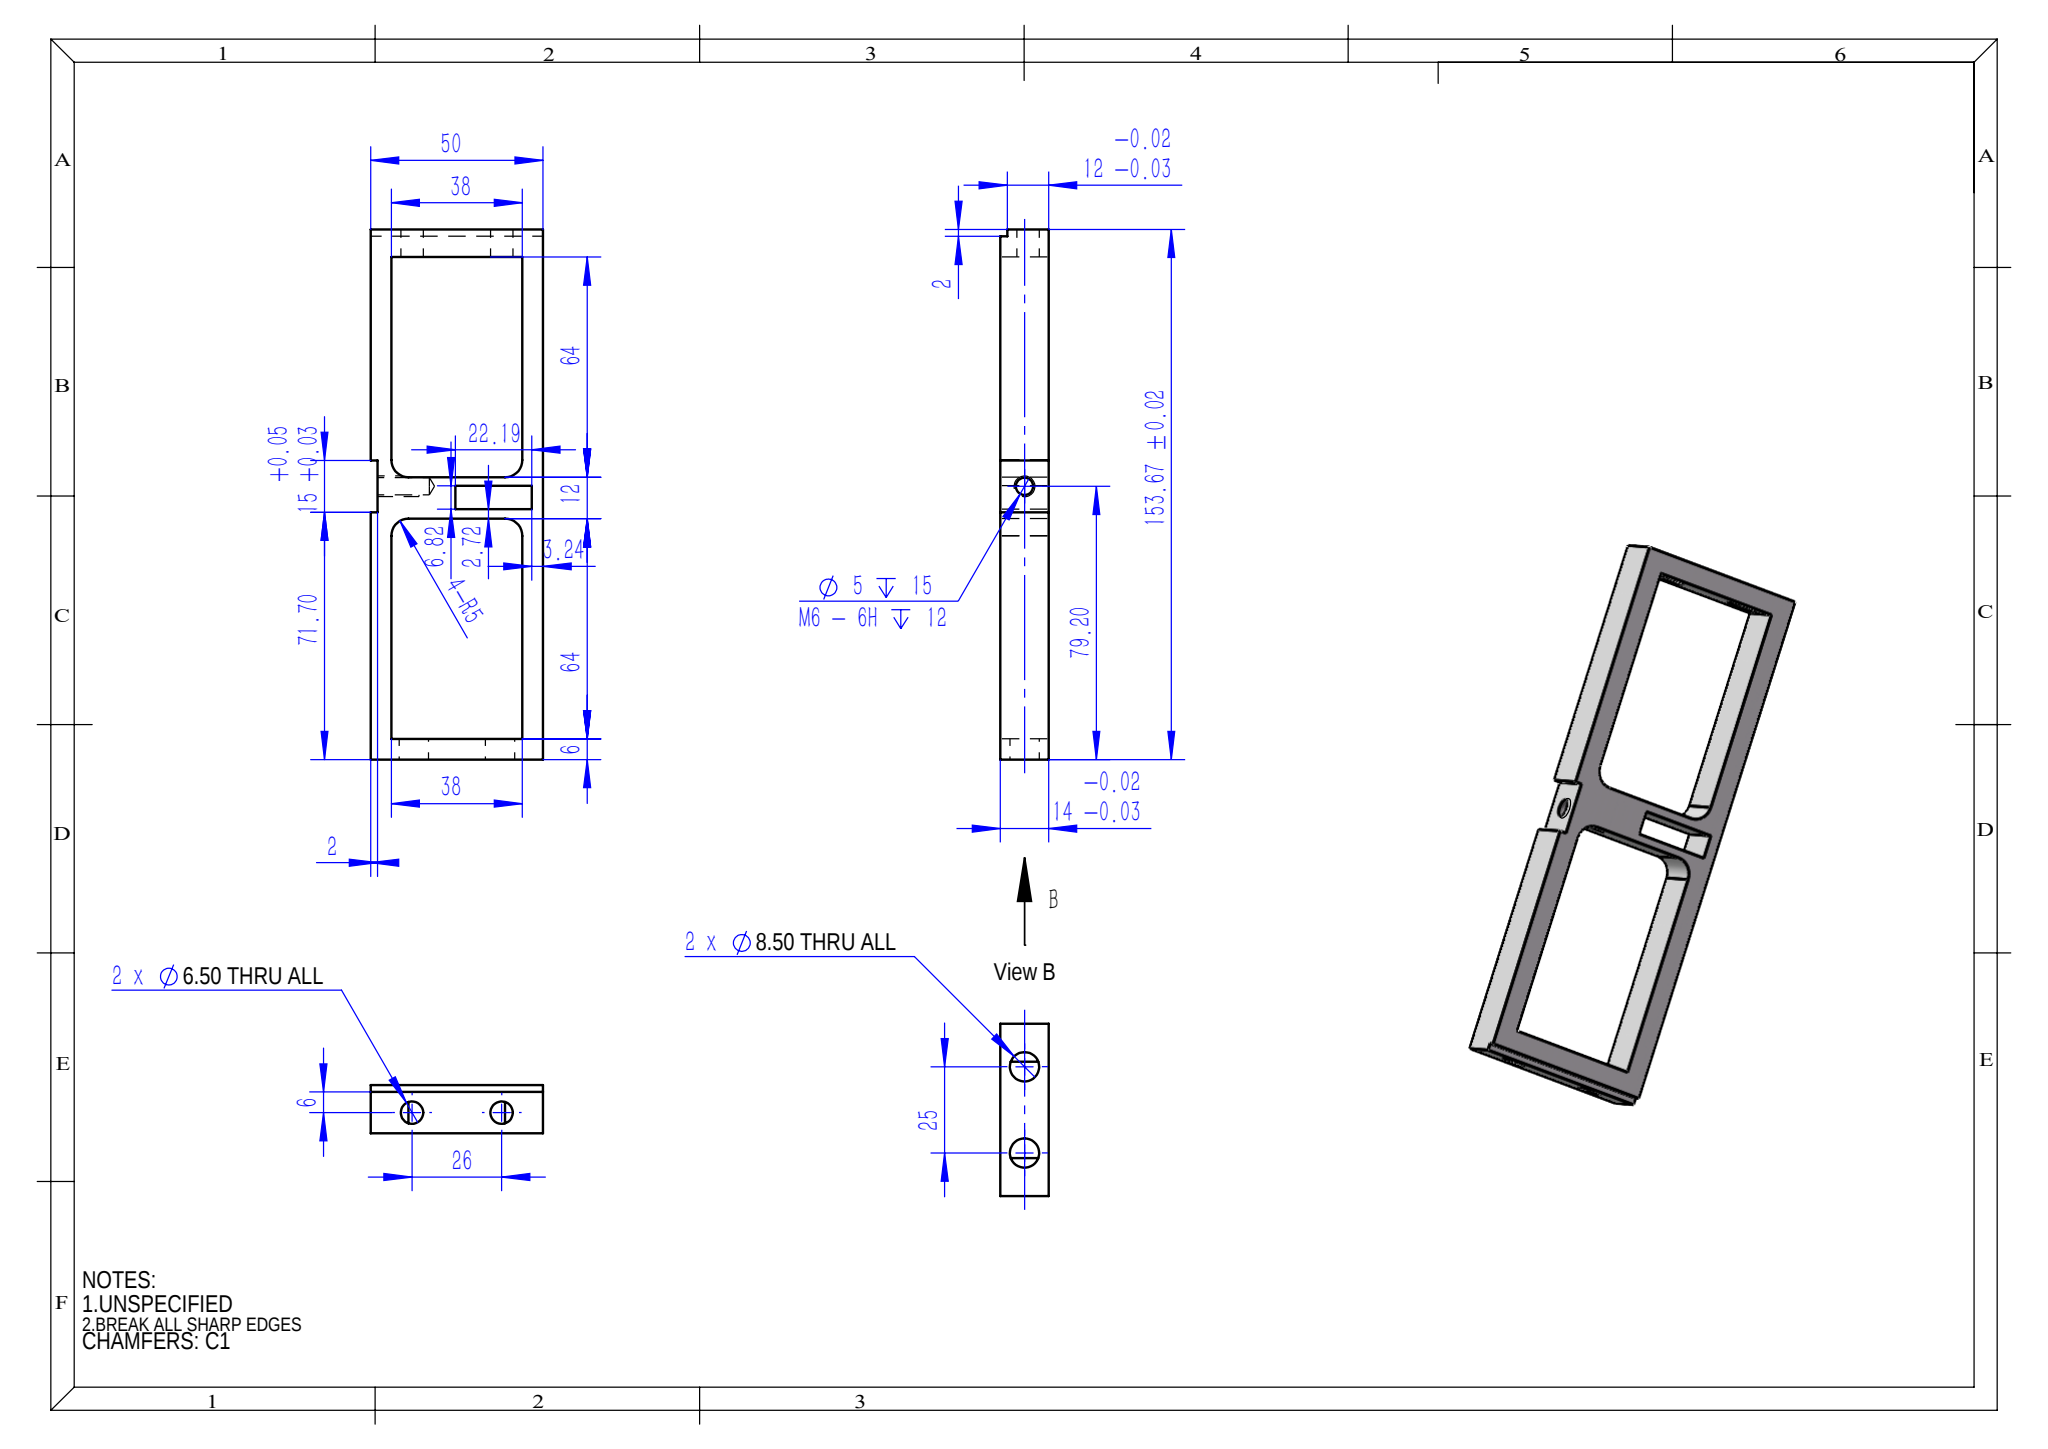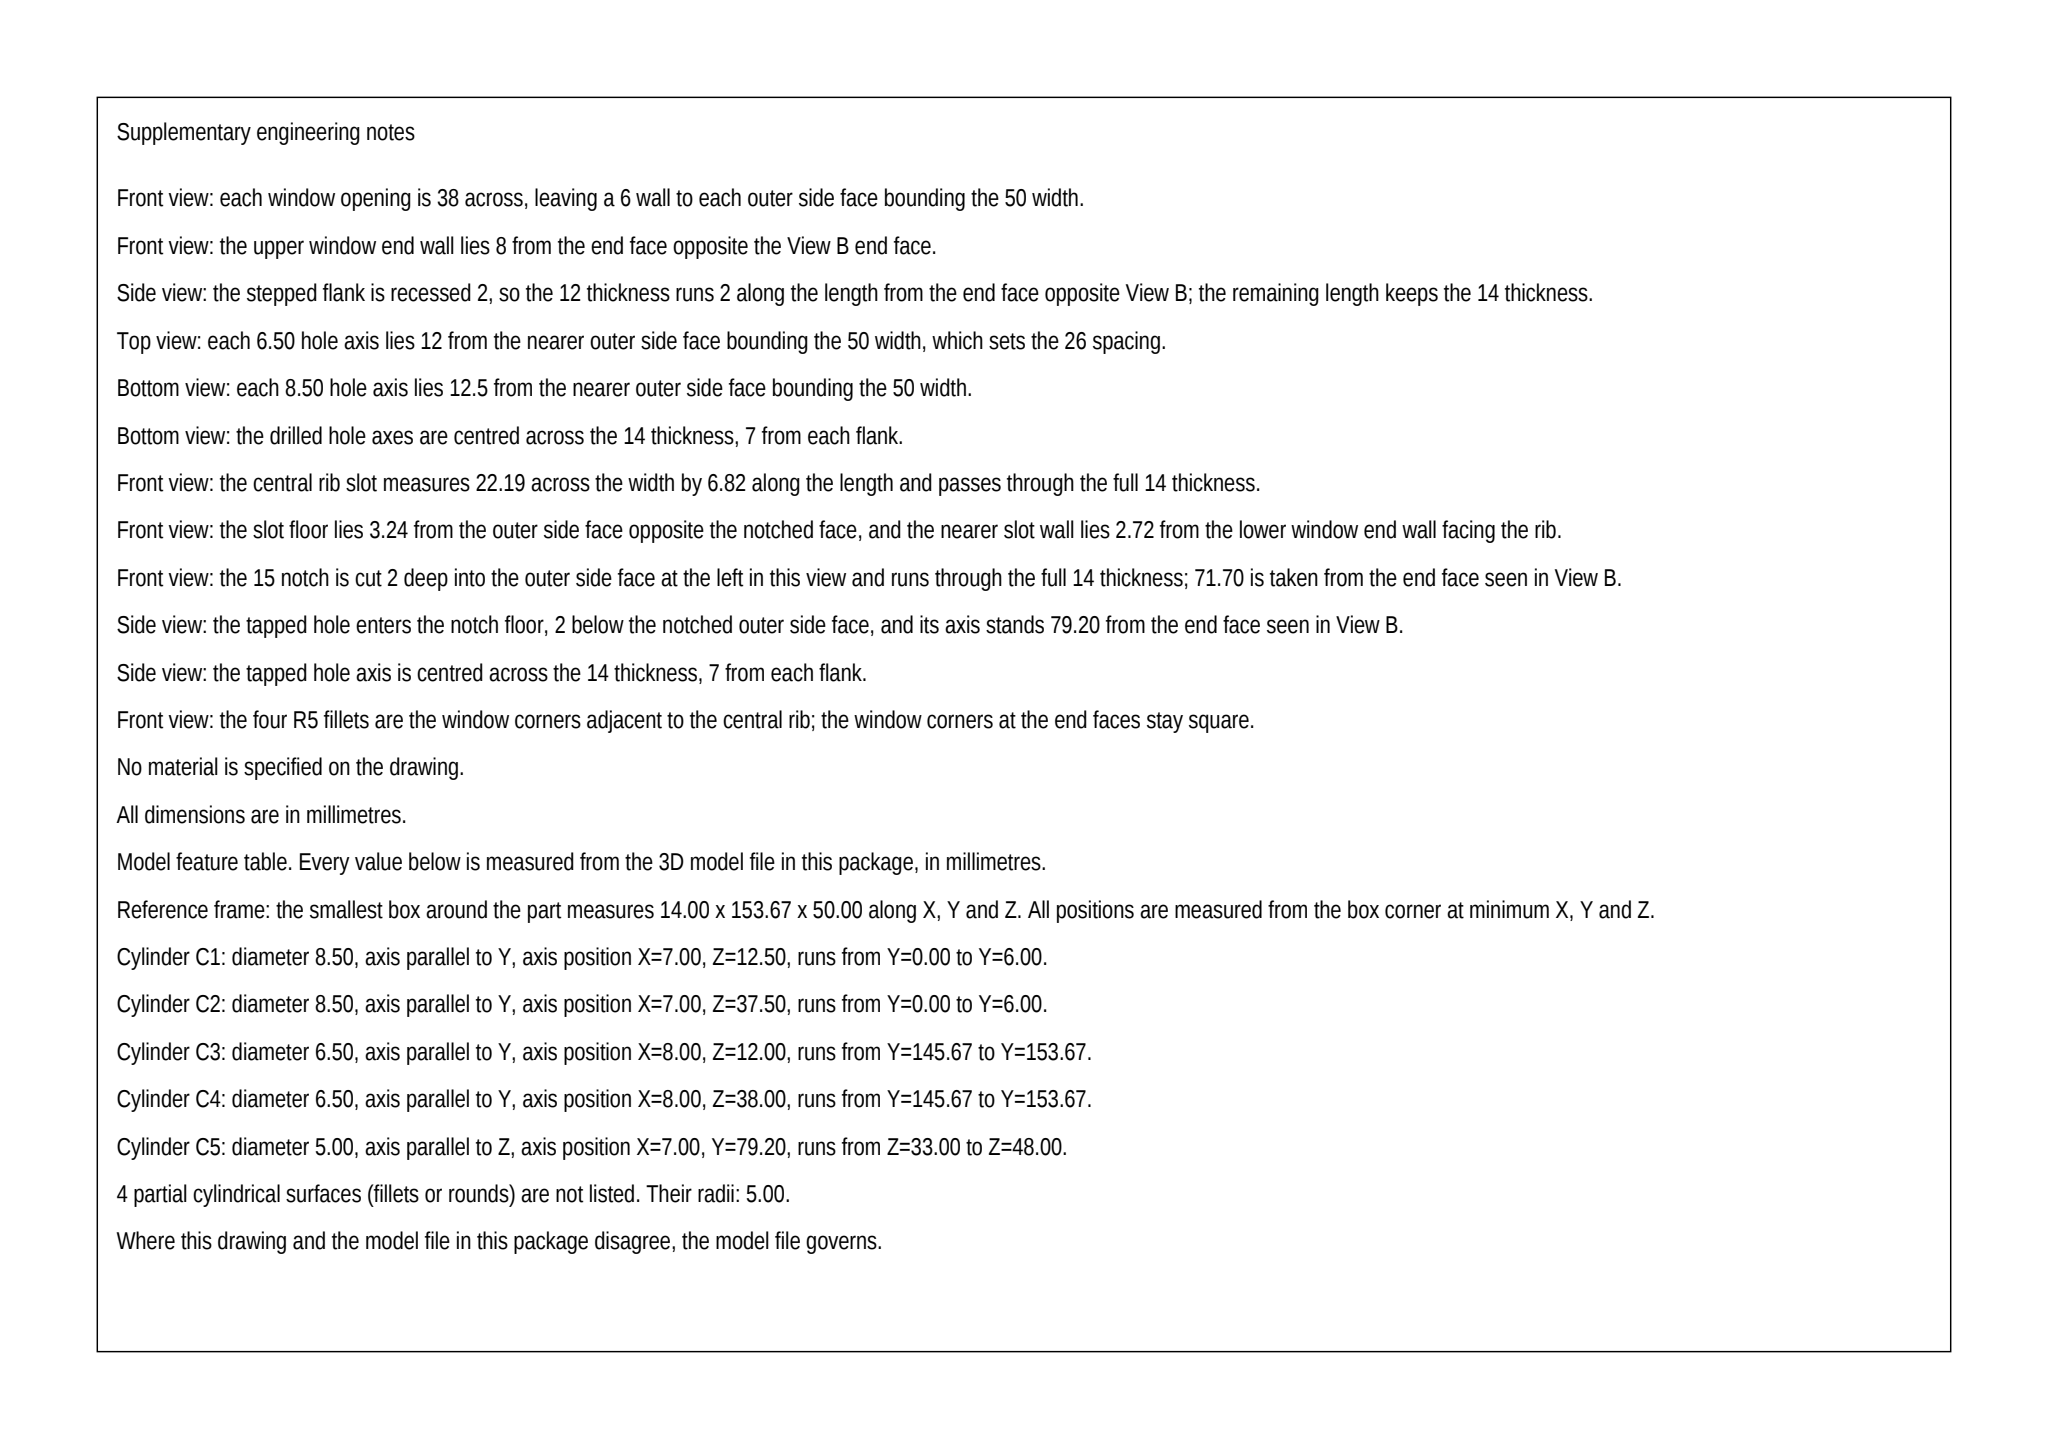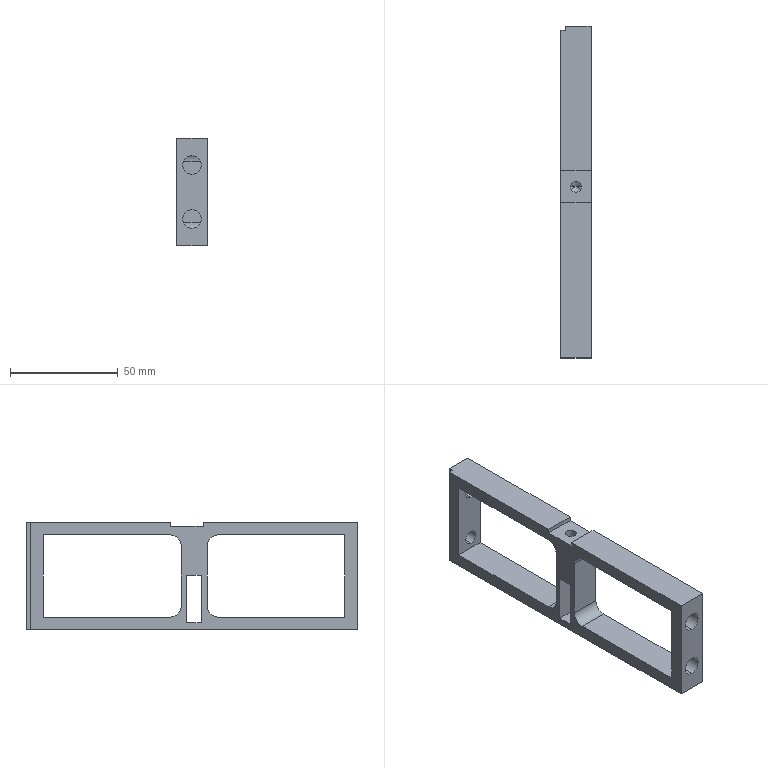Part | SolidWorks | mm | 1 solid | 40 faces | box 14 x 153.67 x 50 mm | volume 35695 mm3 | plane 24 | cylinder 14 | cone 2 | commonest cylinder face diameters 8.5 x4 6.5 x4 10 x4 5 x2
build123d program:
from build123d import *

# Parameters (mm, degrees)
SKETCH1_W                      = 14
SKETCH1_H                      = 153.67
BOSS_EXTRUDE1_DEPTH            = 50
SKETCH15_W                     = 2
SKETCH15_H                     = 2
CUT_EXTRUDE5_DEPTH             = 130.499
SKETCH17_W                     = 38
SKETCH17_H                     = 63.835
CUT_EXTRUDE7_DEPTH             = 129.389
FILLET3_R                      = 5
F_6_5_6_5_DIAMETER_HOLE1_D     = 6.5
F_6_5_6_5_DIAMETER_HOLE1_DEPTH = 8
F_8_5_8_5_DIAMETER_HOLE2_D     = 8.5
F_8_5_8_5_DIAMETER_HOLE2_DEPTH = 6
SKETCH27_W                     = 2
SKETCH27_H                     = 15
CUT_EXTRUDE10_DEPTH            = 129.389
M6_TAPPED_HOLE3_D              = 5
M6_TAPPED_HOLE3_DEPTH          = 15
M6_TAPPED_HOLE3_TIP            = 1.502
SKETCH30_W                     = 22.19
SKETCH30_H                     = 6.818
CUT_EXTRUDE11_DEPTH            = 73


with BuildPart() as part:
    # Sketch1 → Boss-Extrude1 (new body)
    with BuildSketch(Plane.XY):
        with Locations((14.958, 40.587)):
            Rectangle(SKETCH1_W, SKETCH1_H)
    extrude(amount=BOSS_EXTRUDE1_DEPTH)

    # Sketch15 → Cut-Extrude5 (cut, through all)
    with BuildSketch(Plane.XY.offset(50)):
        with Locations((8.958, 116.422)):
            Rectangle(SKETCH15_W, SKETCH15_H)
    extrude(amount=-CUT_EXTRUDE5_DEPTH, mode=Mode.SUBTRACT)

    # Sketch17 → Cut-Extrude7 (cut, through all)
    with BuildSketch(Plane.ZY.offset(-7.958)):
        with Locations((25, 77.504)):
            Rectangle(SKETCH17_W, SKETCH17_H)
        with Locations((25, 1.669)):
            Rectangle(SKETCH17_W, SKETCH17_H)
    extrude(amount=-CUT_EXTRUDE7_DEPTH, mode=Mode.SUBTRACT)

    # Fillet3
    fillet3_edges = [part.edges().sort_by_distance(p)[0] for p in [
        (14.958, 45.587, 6),
        (14.958, 45.587, 44),
        (14.958, 33.587, 6),
        (14.958, 33.587, 44),
    ]]
    fillet(fillet3_edges, radius=FILLET3_R)

    # 6.5 _6.5_ Diameter Hole1
    with Locations(Plane(origin=(0, 109.422, 0), x_dir=(-1, 0, 0), z_dir=(0, -1, 0))):
        with Locations((-15.958, -12), (-15.958, -38)):
            Hole(F_6_5_6_5_DIAMETER_HOLE1_D / 2, depth=F_6_5_6_5_DIAMETER_HOLE1_DEPTH)

    # 8.5 _8.5_ Diameter Hole2
    with Locations(Plane(origin=(0, -30.248, 0), x_dir=(1, 0, 0), z_dir=(0, 1, 0))):
        with Locations((14.958, -37.5), (14.958, -12.5)):
            Hole(F_8_5_8_5_DIAMETER_HOLE2_D / 2, depth=F_8_5_8_5_DIAMETER_HOLE2_DEPTH)

    # Sketch27 → Cut-Extrude10 (cut, through all)
    with BuildSketch(Plane.ZY.offset(-7.958)):
        with Locations((49, 42.952)):
            Rectangle(SKETCH27_W, SKETCH27_H)
    extrude(amount=-CUT_EXTRUDE10_DEPTH, mode=Mode.SUBTRACT)

    # M6 Tapped Hole3
    with Locations(Plane.XY.offset(48)):
        with Locations((14.958, 42.952)):
            Hole(M6_TAPPED_HOLE3_D / 2, depth=M6_TAPPED_HOLE3_DEPTH)
            with Locations((0, 0, -(M6_TAPPED_HOLE3_DEPTH + M6_TAPPED_HOLE3_TIP / 2))):  # 118° drill point
                Cone(0, M6_TAPPED_HOLE3_D / 2, M6_TAPPED_HOLE3_TIP, mode=Mode.SUBTRACT)

    # Sketch30 → Cut-Extrude11 (cut)
    with BuildSketch(Plane.ZY.offset(-7.958)):
        with Locations((14.339, 39.719)):
            Rectangle(SKETCH30_W, SKETCH30_H)
    extrude(amount=-CUT_EXTRUDE11_DEPTH, mode=Mode.SUBTRACT)


solid = part.part